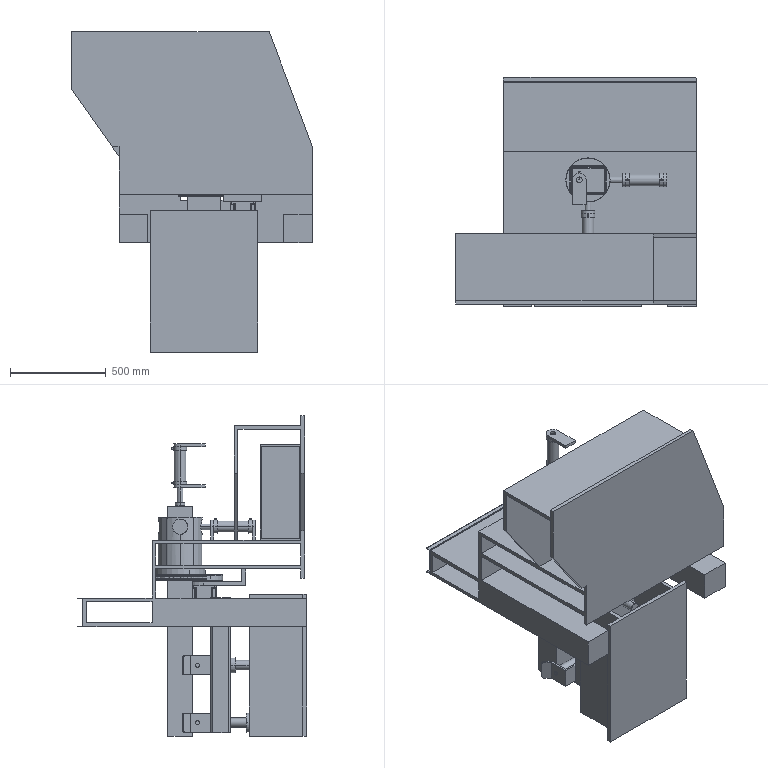Assembly | SolidWorks | mm | 14 component files | 49 solids | 1153 faces | box 1255 x 1197 x 1670.27 mm | volume 200454715 mm3 | cylinder 770 | plane 320 | cone 31 | torus 24 | sphere 8 | commonest cylinder face diameters 7.458 x263 270 x114 264 x113 20 x58 10 x40 2 x28 50 x26 30 x20
Bill of materials:
CoolantTank | 1 | 45 | Plain solid rectangular block (cuboid) with no visible holes, chamfers or features.
HydraulicCylinderA | 1 | 45 | Assembly-like body: a vertical stepped cylinder held between two parallel flat plate arms forming a C/clamp shape; a narrower rod with an end disc sticks out below the lower arm. The upper arm has a rounded end with a through-hole.
HydraulicCylinderB | 1 | 45 | Stepped cylindrical body: a main barrel with larger-diameter collars at each end, a smaller-diameter rod from one end that ends in a disc/flange, and two small radial pin studs on the collars.
HydraulicCylinderC | 2 | 45 | Elongated stepped cylindrical body like unnamed part but longer, carried on two upright plate supports with rounded tops; a smaller rod with an end disc sticks out from one end, and the far support plate has a through-hole.
IdlerRoller | 1 | 45 | Vertical rectangular bar with two long round rods sticking out from one side near the ends, and three bent sheet-style bracket tabs on the opposite side. Each tab has small holes and a short cross pin or roller between its flanges.
IdlerRollerBase | 1 | 45 | Thin-walled open rectangular box or channel made from thin plate: three walls plus a base flange that extends past the walls on both sides, with two small cylindrical bosses on one wall.
MotorMount | 1 | 45 | L-shaped flat tab/bracket: a plate with a semicircular rounded end and a large through-hole, plus a short upturned flange along the opposite straight edge.
Pinion | 1 | 45 | Flat circular disc with a central through-hole and a short coaxial hub boss on one face; edges lightly chamfered.
RotatingSleeve | 1 | 45 | Short cylinder with a square through-cavity along its axis and four cross-holes near one end; small notches at the end edges.
Seat | 1 | 45 | Built-up bracket made of thin plates: a tall angled-profile side plate with a through-hole, joined to horizontal shelf plates and a box-like base, with rectangular bar feet underneath.
ServoMotor130SJT-M075D(AZ) | 1 | Plain Carbon Steel | Square-section body with a square mounting flange that has four corner holes, a raised circular pilot boss, and a central cylindrical shaft with a key/flat feature; the body corners have longitudinal grooves.
SlewingBearing | 1 | 45 | Thin annular ring with a plain cylindrical upper band and a lower band with many fine teeth or knurls around the outside.
Workpiece | 1 | Aviation Aluminum-7075 | Straight, elongated prismatic bar with a rectangular, roughly square cross-section and flat ends; no holes, slots, steps or other features visible.
Mates:
1. distance | Workpiece-1 face at (-5.813, 183.429, 930) dir (1, 0, 0) | HydraulicCylinderA-1 face at (-135.813, 248.429, 930) dir (0, 0, 1) r 25
2. concentric | IdlerRoller-1 face at (-90.813, -311.571, -200) dir (0, 1, 0) r 25 | IdlerRollerBase-1 face at (-90.813, -96.571, -200) dir (0, -1, 0) r 25
3. tangent | Workpiece-1 face at (-5.813, 183.429, 930) dir (0, -1, 0) | IdlerRoller-1 face at (-261.523, 158.429, -200) dir (1, 0, 0) r 25
4. coincident | Workpiece-1 face at (-90.813, 248.429, -270) dir (0, 0, -1) | IdlerRollerBase-1 face at (-90.813, -261.571, -270) dir (0, 0, -1)
5. width | Workpiece-1 face at (-175.813, 183.429, 930) dir (-1, 0, 0) | Workpiece-1 face at (-5.813, 183.429, 930) dir (1, 0, 0) | IdlerRoller-1 face at (-40.813, -1.571, -391.421) dir (1, 0, 0) | IdlerRoller-1 face at (-140.813, -1.571, -391.421) dir (-1, 0, 0)
6. distance | IdlerRollerBase-1 face at (109.187, -111.571, 470) dir (0, 1, 0) | IdlerRoller-1 face at (-50.813, -11.571, -391.421) dir (0, -1, 0)
7. coincident | IdlerRollerBase-1 face at (89.187, -131.571, 470) dir (0, -1, 0) | HydraulicCylinderB-1 face at (-65.813, -131.571, 100) dir (0, 1, 0)
8. concentric | IdlerRollerBase-1 face at (-90.813, -411.572, 100) dir (0, 1, 0) r 50 | HydraulicCylinderB-1 face at (-90.813, -41.571, 100) dir (0, 1, 0) r 25
9. parallel | IdlerRollerBase-1 face at (-90.813, -261.571, 470) dir (0, 0, 1) | HydraulicCylinderB-1 face at (-90.813, -301.571, 185) dir (0, 0, 1)
10. coincident | Seat-1 face at (474.187, -399.571, 602.267) dir (0, 0, -1) | SlewingBearing-1 face at (-90.813, 248.429, 602.267) dir (0, 0, 1)
11. concentric | Seat-1 face at (-90.813, 248.429, 752.267) dir (0, 0, -1) r 115 | SlewingBearing-1 face at (-90.813, 248.429, 572.267) dir (0, 0, 1) r 130
12. concentric | ServoMotor130SJT-M075D(AZ)-1 face at (110.202, 126.699, 572.267) dir (0, 0, -1) r 11 | Pinion-1 face at (110.202, 126.699, 572.267) dir (0, 0, 1) r 11
13. coincident | ServoMotor130SJT-M075D(AZ)-1 face at (110.202, 126.699, 522.267) dir (0, 0, 1) | Pinion-1 face at (102.541, 145.174, 522.267) dir (0, 0, -1)
14. coincident | SlewingBearing-1 face at (-90.813, 248.429, 542.267) dir (0, 0, -1) | Pinion-1 face at (71.897, 219.072, 542.267) dir (0, 0, -1)
15. tangent | SlewingBearing-1 face at (-90.813, 248.429, 542.267) dir (0, 0, 1) r 135 | Pinion-1 face at (110.202, 126.699, 572.267) dir (0, 0, 1) r 100
16. parallel | Seat-1 face at (474.187, 755.429, 450.267) dir (1, 0, 0) | ServoMotor130SJT-M075D(AZ)-1 face at (175.202, 61.699, 514.267) dir (1, 0, 0)
17. concentric | ServoMotor130SJT-M075D(AZ)-1 face at (110.202, 126.699, 520.267) dir (0, 0, -1) r 55 | MotorMount-1 face at (110.202, 126.699, 534.267) dir (0, 0, -1) r 55
18. coincident | ServoMotor130SJT-M075D(AZ)-1 face at (110.202, 126.699, 514.267) dir (0, 0, 1) | MotorMount-1 face at (110.202, 126.699, 514.267) dir (0, 0, -1)
19. parallel | Seat-1 face at (474.187, 755.429, 450.267) dir (1, 0, 0) | MotorMount-1 face at (210.202, -73.301, 534.267) dir (1, 0, 0)
20. concentric | Seat-1 face at (-90.813, 248.429, 752.267) dir (0, 0, -1) r 115 | RotatingSleeve-1 face at (-90.813, 248.429, 872.267) dir (0, 0, -1) r 115
21. coincident | SlewingBearing-1 face at (-90.813, 248.429, 542.267) dir (0, 0, -1) | RotatingSleeve-1 face at (-90.813, 248.429, 542.267) dir (0, 0, -1)
22. concentric | RotatingSleeve-1 face at (24.187, 248.429, 822.267) dir (-1, 0, 0) r 40 | HydraulicCylinderC-1 face at (14.187, 248.429, 822.267) dir (-1, 0, 0) r 15
23. coincident | Workpiece-1 face at (-5.813, 183.429, 930) dir (1, 0, 0) | HydraulicCylinderC-1 face at (-5.813, 248.429, 822.267) dir (-1, 0, 0)
24. parallel | Seat-1 face at (474.187, 395.429, 450.267) dir (0, 1, 0) | HydraulicCylinderC-1 face at (319.187, 283.429, 822.267) dir (0, 1, 0)
25. concentric | RotatingSleeve-1 face at (-90.813, 133.429, 822.267) dir (0, 1, 0) r 40 | HydraulicCylinderC-2 face at (-90.813, 163.429, 822.267) dir (0, 1, 0) r 15
26. coincident | Workpiece-1 face at (-5.813, 183.429, 930) dir (0, -1, 0) | HydraulicCylinderC-2 face at (-90.813, 183.429, 822.267) dir (0, 1, 0)
27. parallel | Seat-1 face at (-533.813, 755.429, 450.267) dir (-1, 0, 0) | HydraulicCylinderC-2 face at (-125.813, 88.429, 752.267) dir (-1, 0, 0)
28. coincident | Seat-1 face at (-533.813, -379.571, 802.267) dir (0, 1, 0) | CoolantTank-1 face at (145.187, -379.571, 1252.267) dir (0, -1, 0)
29. coincident | Seat-1 face at (474.187, 395.429, 752.267) dir (0, 0, 1) | CoolantTank-1 face at (-84.813, -274.571, 752.267) dir (0, 0, -1)
30. width | Seat-1 face at (124.187, -399.572, 752.267) dir (-1, 0, 0) | Seat-1 face at (-293.813, -399.572, 752.267) dir (1, 0, 0) | CoolantTank-1 face at (-319.813, -374.571, 1252.267) dir (-1, 0, 0) | CoolantTank-1 face at (150.187, -374.571, 1252.267) dir (1, 0, 0)